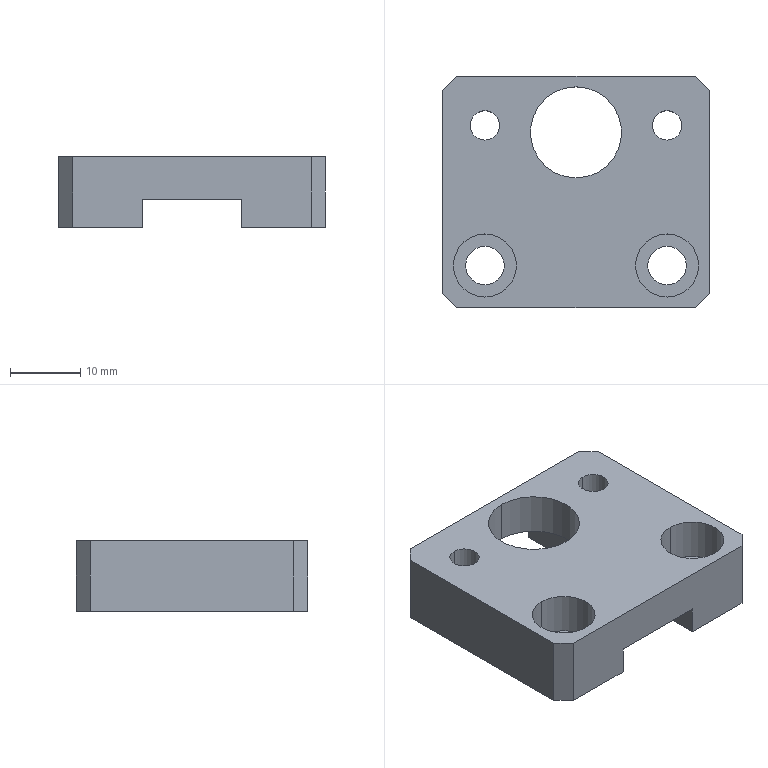Component | SolidWorks | DZ.KX.203-TC1505-30-09-01-05-19-1 | 1 solid | 30 faces | box 38 x 33 x 10 mm | volume 8585 mm3 | plane 16 | cylinder 14 | commonest cylinder face diameters 9 x4 5.5 x4 4.2 x4 13 x2
STEP:
#1=CARTESIAN_POINT('',(11.083,-23.614,0.8291));
#2=VERTEX_POINT('',#1);
#3=CARTESIAN_POINT('',(11.083,-23.26,0.8291));
#4=VERTEX_POINT('',#3);
#5=CARTESIAN_POINT('',(11.083,-23.437,0.8291));
#6=DIRECTION('',(0.,0.,1.));
#7=DIRECTION('',(0.,1.,0.));
#8=AXIS2_PLACEMENT_3D('',#5,#6,#7);
#9=CIRCLE('',#8,0.1772);
#10=EDGE_CURVE('',#2,#4,#9,.T.);
#11=ORIENTED_EDGE('',*,*,#10,.F.);
#12=CARTESIAN_POINT('',(11.083,-23.614,1.065));
#13=VERTEX_POINT('',#12);
#14=CARTESIAN_POINT('',(11.083,-23.614,1.065));
#15=DIRECTION('',(0.,0.,1.));
#16=VECTOR('',#15,39.37);
#17=LINE('',#14,#16);
#18=EDGE_CURVE('',#2,#13,#17,.T.);
#19=ORIENTED_EDGE('',*,*,#18,.T.);
#20=CARTESIAN_POINT('',(11.083,-23.26,1.065));
#21=VERTEX_POINT('',#20);
#22=CARTESIAN_POINT('',(11.083,-23.437,1.065));
#23=DIRECTION('',(0.,0.,1.));
#24=DIRECTION('',(0.,1.,0.));
#25=AXIS2_PLACEMENT_3D('',#22,#23,#24);
#26=CIRCLE('',#25,0.1772);
#27=EDGE_CURVE('',#13,#21,#26,.T.);
#28=ORIENTED_EDGE('',*,*,#27,.T.);
#29=CARTESIAN_POINT('',(11.083,-23.26,1.065));
#30=DIRECTION('',(0.,0.,1.));
#31=VECTOR('',#30,39.37);
#32=LINE('',#29,#31);
#33=EDGE_CURVE('',#4,#21,#32,.T.);
#34=ORIENTED_EDGE('',*,*,#33,.F.);
#35=EDGE_LOOP('',(#11,#19,#28,#34));
#36=FACE_OUTER_BOUND('',#35,.T.);
#37=CARTESIAN_POINT('',(11.083,-23.437,1.065));
#38=DIRECTION('',(0.,0.,1.));
#39=DIRECTION('',(0.,1.,0.));
#40=AXIS2_PLACEMENT_3D('',#37,#38,#39);
#41=CYLINDRICAL_SURFACE('',#40,0.1772);
#42=ADVANCED_FACE('',(#36),#41,.F.);
#43=CARTESIAN_POINT('',(11.083,-23.329,0.6716));
#44=VERTEX_POINT('',#43);
#45=CARTESIAN_POINT('',(11.083,-23.546,0.6716));
#46=VERTEX_POINT('',#45);
#47=CARTESIAN_POINT('',(11.083,-23.437,0.6716));
#48=DIRECTION('',(-0.,-0.,-1.));
#49=DIRECTION('',(0.,-1.,0.));
#50=AXIS2_PLACEMENT_3D('',#47,#48,#49);
#51=CIRCLE('',#50,0.1083);
#52=EDGE_CURVE('',#44,#46,#51,.T.);
#53=ORIENTED_EDGE('',*,*,#52,.T.);
#54=CARTESIAN_POINT('',(11.083,-23.546,0.8291));
#55=VERTEX_POINT('',#54);
#56=CARTESIAN_POINT('',(11.083,-23.546,1.065));
#57=DIRECTION('',(0.,0.,1.));
#58=VECTOR('',#57,39.37);
#59=LINE('',#56,#58);
#60=EDGE_CURVE('',#46,#55,#59,.T.);
#61=ORIENTED_EDGE('',*,*,#60,.T.);
#62=CARTESIAN_POINT('',(11.083,-23.329,0.8291));
#63=VERTEX_POINT('',#62);
#64=CARTESIAN_POINT('',(11.083,-23.437,0.8291));
#65=DIRECTION('',(0.,0.,1.));
#66=DIRECTION('',(0.,1.,0.));
#67=AXIS2_PLACEMENT_3D('',#64,#65,#66);
#68=CIRCLE('',#67,0.1083);
#69=EDGE_CURVE('',#55,#63,#68,.T.);
#70=ORIENTED_EDGE('',*,*,#69,.T.);
#71=CARTESIAN_POINT('',(11.083,-23.329,1.065));
#72=DIRECTION('',(0.,0.,1.));
#73=VECTOR('',#72,39.37);
#74=LINE('',#71,#73);
#75=EDGE_CURVE('',#44,#63,#74,.T.);
#76=ORIENTED_EDGE('',*,*,#75,.F.);
#77=EDGE_LOOP('',(#53,#61,#70,#76));
#78=FACE_OUTER_BOUND('',#77,.T.);
#79=CARTESIAN_POINT('',(11.083,-23.437,1.065));
#80=DIRECTION('',(0.,0.,1.));
#81=DIRECTION('',(0.,1.,0.));
#82=AXIS2_PLACEMENT_3D('',#79,#80,#81);
#83=CYLINDRICAL_SURFACE('',#82,0.1083);
#84=ADVANCED_FACE('',(#78),#83,.F.);
#85=CARTESIAN_POINT('',(12.106,-23.614,0.8291));
#86=VERTEX_POINT('',#85);
#87=CARTESIAN_POINT('',(12.106,-23.26,0.8291));
#88=VERTEX_POINT('',#87);
#89=CARTESIAN_POINT('',(12.106,-23.437,0.8291));
#90=DIRECTION('',(0.,0.,1.));
#91=DIRECTION('',(0.,1.,0.));
#92=AXIS2_PLACEMENT_3D('',#89,#90,#91);
#93=CIRCLE('',#92,0.1772);
#94=EDGE_CURVE('',#86,#88,#93,.T.);
#95=ORIENTED_EDGE('',*,*,#94,.F.);
#96=CARTESIAN_POINT('',(12.106,-23.614,1.065));
#97=VERTEX_POINT('',#96);
#98=CARTESIAN_POINT('',(12.106,-23.614,1.065));
#99=DIRECTION('',(0.,0.,1.));
#100=VECTOR('',#99,39.37);
#101=LINE('',#98,#100);
#102=EDGE_CURVE('',#86,#97,#101,.T.);
#103=ORIENTED_EDGE('',*,*,#102,.T.);
#104=CARTESIAN_POINT('',(12.106,-23.26,1.065));
#105=VERTEX_POINT('',#104);
#106=CARTESIAN_POINT('',(12.106,-23.437,1.065));
#107=DIRECTION('',(0.,0.,1.));
#108=DIRECTION('',(0.,1.,0.));
#109=AXIS2_PLACEMENT_3D('',#106,#107,#108);
#110=CIRCLE('',#109,0.1772);
#111=EDGE_CURVE('',#97,#105,#110,.T.);
#112=ORIENTED_EDGE('',*,*,#111,.T.);
#113=CARTESIAN_POINT('',(12.106,-23.26,1.065));
#114=DIRECTION('',(0.,0.,1.));
#115=VECTOR('',#114,39.37);
#116=LINE('',#113,#115);
#117=EDGE_CURVE('',#88,#105,#116,.T.);
#118=ORIENTED_EDGE('',*,*,#117,.F.);
#119=EDGE_LOOP('',(#95,#103,#112,#118));
#120=FACE_OUTER_BOUND('',#119,.T.);
#121=CARTESIAN_POINT('',(12.106,-23.437,1.065));
#122=DIRECTION('',(0.,0.,1.));
#123=DIRECTION('',(0.,1.,0.));
#124=AXIS2_PLACEMENT_3D('',#121,#122,#123);
#125=CYLINDRICAL_SURFACE('',#124,0.1772);
#126=ADVANCED_FACE('',(#120),#125,.F.);
#127=CARTESIAN_POINT('',(12.106,-23.329,0.6716));
#128=VERTEX_POINT('',#127);
#129=CARTESIAN_POINT('',(12.106,-23.546,0.6716));
#130=VERTEX_POINT('',#129);
#131=CARTESIAN_POINT('',(12.106,-23.437,0.6716));
#132=DIRECTION('',(-0.,-0.,-1.));
#133=DIRECTION('',(0.,-1.,0.));
#134=AXIS2_PLACEMENT_3D('',#131,#132,#133);
#135=CIRCLE('',#134,0.1083);
#136=EDGE_CURVE('',#128,#130,#135,.T.);
#137=ORIENTED_EDGE('',*,*,#136,.T.);
#138=CARTESIAN_POINT('',(12.106,-23.546,0.8291));
#139=VERTEX_POINT('',#138);
#140=CARTESIAN_POINT('',(12.106,-23.546,1.065));
#141=DIRECTION('',(0.,0.,1.));
#142=VECTOR('',#141,39.37);
#143=LINE('',#140,#142);
#144=EDGE_CURVE('',#130,#139,#143,.T.);
#145=ORIENTED_EDGE('',*,*,#144,.T.);
#146=CARTESIAN_POINT('',(12.106,-23.329,0.8291));
#147=VERTEX_POINT('',#146);
#148=CARTESIAN_POINT('',(12.106,-23.437,0.8291));
#149=DIRECTION('',(0.,0.,1.));
#150=DIRECTION('',(0.,1.,0.));
#151=AXIS2_PLACEMENT_3D('',#148,#149,#150);
#152=CIRCLE('',#151,0.1083);
#153=EDGE_CURVE('',#139,#147,#152,.T.);
#154=ORIENTED_EDGE('',*,*,#153,.T.);
#155=CARTESIAN_POINT('',(12.106,-23.329,1.065));
#156=DIRECTION('',(0.,0.,1.));
#157=VECTOR('',#156,39.37);
#158=LINE('',#155,#157);
#159=EDGE_CURVE('',#128,#147,#158,.T.);
#160=ORIENTED_EDGE('',*,*,#159,.F.);
#161=EDGE_LOOP('',(#137,#145,#154,#160));
#162=FACE_OUTER_BOUND('',#161,.T.);
#163=CARTESIAN_POINT('',(12.106,-23.437,1.065));
#164=DIRECTION('',(0.,0.,1.));
#165=DIRECTION('',(0.,1.,0.));
#166=AXIS2_PLACEMENT_3D('',#163,#164,#165);
#167=CYLINDRICAL_SURFACE('',#166,0.1083);
#168=ADVANCED_FACE('',(#162),#167,.F.);
#169=CARTESIAN_POINT('',(11.083,-22.567,1.065));
#170=VERTEX_POINT('',#169);
#171=CARTESIAN_POINT('',(11.083,-22.733,1.065));
#172=VERTEX_POINT('',#171);
#173=CARTESIAN_POINT('',(11.083,-22.65,1.065));
#174=DIRECTION('',(-0.,-0.,-1.));
#175=DIRECTION('',(0.,-1.,0.));
#176=AXIS2_PLACEMENT_3D('',#173,#174,#175);
#177=CIRCLE('',#176,0.08268);
#178=EDGE_CURVE('',#170,#172,#177,.T.);
#179=ORIENTED_EDGE('',*,*,#178,.F.);
#180=CARTESIAN_POINT('',(11.083,-22.567,0.6716));
#181=VERTEX_POINT('',#180);
#182=CARTESIAN_POINT('',(11.083,-22.567,0.6716));
#183=DIRECTION('',(-0.,-0.,-1.));
#184=VECTOR('',#183,39.37);
#185=LINE('',#182,#184);
#186=EDGE_CURVE('',#170,#181,#185,.T.);
#187=ORIENTED_EDGE('',*,*,#186,.T.);
#188=CARTESIAN_POINT('',(11.083,-22.733,0.6716));
#189=VERTEX_POINT('',#188);
#190=CARTESIAN_POINT('',(11.083,-22.65,0.6716));
#191=DIRECTION('',(-0.,-0.,-1.));
#192=DIRECTION('',(0.,-1.,0.));
#193=AXIS2_PLACEMENT_3D('',#190,#191,#192);
#194=CIRCLE('',#193,0.08268);
#195=EDGE_CURVE('',#181,#189,#194,.T.);
#196=ORIENTED_EDGE('',*,*,#195,.T.);
#197=CARTESIAN_POINT('',(11.083,-22.733,0.6716));
#198=DIRECTION('',(-0.,-0.,-1.));
#199=VECTOR('',#198,39.37);
#200=LINE('',#197,#199);
#201=EDGE_CURVE('',#172,#189,#200,.T.);
#202=ORIENTED_EDGE('',*,*,#201,.F.);
#203=EDGE_LOOP('',(#179,#187,#196,#202));
#204=FACE_OUTER_BOUND('',#203,.T.);
#205=CARTESIAN_POINT('',(11.083,-22.65,0.6716));
#206=DIRECTION('',(-0.,-0.,-1.));
#207=DIRECTION('',(0.,-1.,0.));
#208=AXIS2_PLACEMENT_3D('',#205,#206,#207);
#209=CYLINDRICAL_SURFACE('',#208,0.08268);
#210=ADVANCED_FACE('',(#204),#209,.F.);
#211=CARTESIAN_POINT('',(12.106,-22.567,1.065));
#212=VERTEX_POINT('',#211);
#213=CARTESIAN_POINT('',(12.106,-22.733,1.065));
#214=VERTEX_POINT('',#213);
#215=CARTESIAN_POINT('',(12.106,-22.65,1.065));
#216=DIRECTION('',(-0.,-0.,-1.));
#217=DIRECTION('',(0.,-1.,0.));
#218=AXIS2_PLACEMENT_3D('',#215,#216,#217);
#219=CIRCLE('',#218,0.08268);
#220=EDGE_CURVE('',#212,#214,#219,.T.);
#221=ORIENTED_EDGE('',*,*,#220,.F.);
#222=CARTESIAN_POINT('',(12.106,-22.567,0.6716));
#223=VERTEX_POINT('',#222);
#224=CARTESIAN_POINT('',(12.106,-22.567,0.6716));
#225=DIRECTION('',(-0.,-0.,-1.));
#226=VECTOR('',#225,39.37);
#227=LINE('',#224,#226);
#228=EDGE_CURVE('',#212,#223,#227,.T.);
#229=ORIENTED_EDGE('',*,*,#228,.T.);
#230=CARTESIAN_POINT('',(12.106,-22.733,0.6716));
#231=VERTEX_POINT('',#230);
#232=CARTESIAN_POINT('',(12.106,-22.65,0.6716));
#233=DIRECTION('',(-0.,-0.,-1.));
#234=DIRECTION('',(0.,-1.,0.));
#235=AXIS2_PLACEMENT_3D('',#232,#233,#234);
#236=CIRCLE('',#235,0.08268);
#237=EDGE_CURVE('',#223,#231,#236,.T.);
#238=ORIENTED_EDGE('',*,*,#237,.T.);
#239=CARTESIAN_POINT('',(12.106,-22.733,0.6716));
#240=DIRECTION('',(-0.,-0.,-1.));
#241=VECTOR('',#240,39.37);
#242=LINE('',#239,#241);
#243=EDGE_CURVE('',#214,#231,#242,.T.);
#244=ORIENTED_EDGE('',*,*,#243,.F.);
#245=EDGE_LOOP('',(#221,#229,#238,#244));
#246=FACE_OUTER_BOUND('',#245,.T.);
#247=CARTESIAN_POINT('',(12.106,-22.65,0.6716));
#248=DIRECTION('',(-0.,-0.,-1.));
#249=DIRECTION('',(0.,-1.,0.));
#250=AXIS2_PLACEMENT_3D('',#247,#248,#249);
#251=CYLINDRICAL_SURFACE('',#250,0.08268);
#252=ADVANCED_FACE('',(#246),#251,.F.);
#253=CARTESIAN_POINT('',(11.594,-22.433,0.8291));
#254=VERTEX_POINT('',#253);
#255=CARTESIAN_POINT('',(11.594,-22.945,0.8291));
#256=VERTEX_POINT('',#255);
#257=CARTESIAN_POINT('',(11.594,-22.689,0.8291));
#258=DIRECTION('',(-0.,-0.,-1.));
#259=DIRECTION('',(0.,-1.,0.));
#260=AXIS2_PLACEMENT_3D('',#257,#258,#259);
#261=CIRCLE('',#260,0.2559);
#262=EDGE_CURVE('',#254,#256,#261,.T.);
#263=ORIENTED_EDGE('',*,*,#262,.T.);
#264=CARTESIAN_POINT('',(11.594,-22.945,1.065));
#265=VERTEX_POINT('',#264);
#266=CARTESIAN_POINT('',(11.594,-22.945,0.6716));
#267=DIRECTION('',(0.,0.,1.));
#268=VECTOR('',#267,39.37);
#269=LINE('',#266,#268);
#270=EDGE_CURVE('',#256,#265,#269,.T.);
#271=ORIENTED_EDGE('',*,*,#270,.T.);
#272=CARTESIAN_POINT('',(11.594,-22.433,1.065));
#273=VERTEX_POINT('',#272);
#274=CARTESIAN_POINT('',(11.594,-22.689,1.065));
#275=DIRECTION('',(-0.,-0.,-1.));
#276=DIRECTION('',(0.,-1.,0.));
#277=AXIS2_PLACEMENT_3D('',#274,#275,#276);
#278=CIRCLE('',#277,0.2559);
#279=EDGE_CURVE('',#273,#265,#278,.T.);
#280=ORIENTED_EDGE('',*,*,#279,.F.);
#281=CARTESIAN_POINT('',(11.594,-22.433,0.6716));
#282=DIRECTION('',(0.,0.,1.));
#283=VECTOR('',#282,39.37);
#284=LINE('',#281,#283);
#285=EDGE_CURVE('',#254,#273,#284,.T.);
#286=ORIENTED_EDGE('',*,*,#285,.F.);
#287=EDGE_LOOP('',(#263,#271,#280,#286));
#288=FACE_OUTER_BOUND('',#287,.T.);
#289=CARTESIAN_POINT('',(11.594,-22.689,0.6716));
#290=DIRECTION('',(0.,0.,1.));
#291=DIRECTION('',(0.,1.,0.));
#292=AXIS2_PLACEMENT_3D('',#289,#290,#291);
#293=CYLINDRICAL_SURFACE('',#292,0.2559);
#294=ADVANCED_FACE('',(#288),#293,.F.);
#295=CARTESIAN_POINT('',(11.083,-23.437,1.065));
#296=DIRECTION('',(0.,0.,1.));
#297=DIRECTION('',(0.,1.,0.));
#298=AXIS2_PLACEMENT_3D('',#295,#296,#297);
#299=CIRCLE('',#298,0.1772);
#300=EDGE_CURVE('',#21,#13,#299,.T.);
#301=ORIENTED_EDGE('',*,*,#300,.F.);
#302=ORIENTED_EDGE('',*,*,#27,.F.);
#303=EDGE_LOOP('',(#301,#302));
#304=FACE_BOUND('',#303,.T.);
#305=CARTESIAN_POINT('',(12.106,-23.437,1.065));
#306=DIRECTION('',(0.,0.,1.));
#307=DIRECTION('',(0.,1.,0.));
#308=AXIS2_PLACEMENT_3D('',#305,#306,#307);
#309=CIRCLE('',#308,0.1772);
#310=EDGE_CURVE('',#105,#97,#309,.T.);
#311=ORIENTED_EDGE('',*,*,#310,.F.);
#312=ORIENTED_EDGE('',*,*,#111,.F.);
#313=EDGE_LOOP('',(#311,#312));
#314=FACE_BOUND('',#313,.T.);
#315=CARTESIAN_POINT('',(11.083,-22.65,1.065));
#316=DIRECTION('',(-0.,-0.,-1.));
#317=DIRECTION('',(0.,-1.,0.));
#318=AXIS2_PLACEMENT_3D('',#315,#316,#317);
#319=CIRCLE('',#318,0.08268);
#320=EDGE_CURVE('',#172,#170,#319,.T.);
#321=ORIENTED_EDGE('',*,*,#320,.T.);
#322=ORIENTED_EDGE('',*,*,#178,.T.);
#323=EDGE_LOOP('',(#321,#322));
#324=FACE_BOUND('',#323,.T.);
#325=CARTESIAN_POINT('',(12.106,-22.65,1.065));
#326=DIRECTION('',(-0.,-0.,-1.));
#327=DIRECTION('',(0.,-1.,0.));
#328=AXIS2_PLACEMENT_3D('',#325,#326,#327);
#329=CIRCLE('',#328,0.08268);
#330=EDGE_CURVE('',#214,#212,#329,.T.);
#331=ORIENTED_EDGE('',*,*,#330,.T.);
#332=ORIENTED_EDGE('',*,*,#220,.T.);
#333=EDGE_LOOP('',(#331,#332));
#334=FACE_BOUND('',#333,.T.);
#335=CARTESIAN_POINT('',(12.264,-23.674,1.065));
#336=VERTEX_POINT('',#335);
#337=CARTESIAN_POINT('',(10.925,-23.674,1.065));
#338=VERTEX_POINT('',#337);
#339=CARTESIAN_POINT('',(12.264,-23.674,1.065));
#340=DIRECTION('',(-1.,-0.,0.));
#341=VECTOR('',#340,39.37);
#342=LINE('',#339,#341);
#343=EDGE_CURVE('',#336,#338,#342,.T.);
#344=ORIENTED_EDGE('',*,*,#343,.F.);
#345=CARTESIAN_POINT('',(12.343,-23.595,1.065));
#346=VERTEX_POINT('',#345);
#347=CARTESIAN_POINT('',(12.264,-23.674,1.065));
#348=DIRECTION('',(0.7071,0.7071,-0.));
#349=VECTOR('',#348,39.37);
#350=LINE('',#347,#349);
#351=EDGE_CURVE('',#336,#346,#350,.T.);
#352=ORIENTED_EDGE('',*,*,#351,.T.);
#353=CARTESIAN_POINT('',(12.343,-22.453,1.065));
#354=VERTEX_POINT('',#353);
#355=CARTESIAN_POINT('',(12.343,-22.453,1.065));
#356=DIRECTION('',(0.,-1.,0.));
#357=VECTOR('',#356,39.37);
#358=LINE('',#355,#357);
#359=EDGE_CURVE('',#354,#346,#358,.T.);
#360=ORIENTED_EDGE('',*,*,#359,.F.);
#361=CARTESIAN_POINT('',(12.264,-22.374,1.065));
#362=VERTEX_POINT('',#361);
#363=CARTESIAN_POINT('',(12.264,-22.374,1.065));
#364=DIRECTION('',(0.7071,-0.7071,-0.));
#365=VECTOR('',#364,39.37);
#366=LINE('',#363,#365);
#367=EDGE_CURVE('',#362,#354,#366,.T.);
#368=ORIENTED_EDGE('',*,*,#367,.F.);
#369=CARTESIAN_POINT('',(10.925,-22.374,1.065));
#370=VERTEX_POINT('',#369);
#371=CARTESIAN_POINT('',(10.925,-22.374,1.065));
#372=DIRECTION('',(1.,0.,-0.));
#373=VECTOR('',#372,39.37);
#374=LINE('',#371,#373);
#375=EDGE_CURVE('',#370,#362,#374,.T.);
#376=ORIENTED_EDGE('',*,*,#375,.F.);
#377=CARTESIAN_POINT('',(10.846,-22.453,1.065));
#378=VERTEX_POINT('',#377);
#379=CARTESIAN_POINT('',(10.846,-22.453,1.065));
#380=DIRECTION('',(0.7071,0.7071,-0.));
#381=VECTOR('',#380,39.37);
#382=LINE('',#379,#381);
#383=EDGE_CURVE('',#378,#370,#382,.T.);
#384=ORIENTED_EDGE('',*,*,#383,.F.);
#385=CARTESIAN_POINT('',(10.846,-23.595,1.065));
#386=VERTEX_POINT('',#385);
#387=CARTESIAN_POINT('',(10.846,-22.925,1.065));
#388=DIRECTION('',(-0.,1.,-0.));
#389=VECTOR('',#388,39.37);
#390=LINE('',#387,#389);
#391=EDGE_CURVE('',#386,#378,#390,.T.);
#392=ORIENTED_EDGE('',*,*,#391,.F.);
#393=CARTESIAN_POINT('',(10.846,-23.595,1.065));
#394=DIRECTION('',(0.7071,-0.7071,-0.));
#395=VECTOR('',#394,39.37);
#396=LINE('',#393,#395);
#397=EDGE_CURVE('',#386,#338,#396,.T.);
#398=ORIENTED_EDGE('',*,*,#397,.T.);
#399=EDGE_LOOP('',(#344,#352,#360,#368,#376,#384,#392,#398));
#400=FACE_OUTER_BOUND('',#399,.T.);
#401=ORIENTED_EDGE('',*,*,#279,.T.);
#402=CARTESIAN_POINT('',(11.594,-22.689,1.065));
#403=DIRECTION('',(-0.,-0.,-1.));
#404=DIRECTION('',(0.,-1.,0.));
#405=AXIS2_PLACEMENT_3D('',#402,#403,#404);
#406=CIRCLE('',#405,0.2559);
#407=EDGE_CURVE('',#265,#273,#406,.T.);
#408=ORIENTED_EDGE('',*,*,#407,.T.);
#409=EDGE_LOOP('',(#401,#408));
#410=FACE_BOUND('',#409,.T.);
#411=CARTESIAN_POINT('',(12.343,-22.374,1.065));
#412=DIRECTION('',(-0.,-0.,-1.));
#413=DIRECTION('',(0.,-1.,0.));
#414=AXIS2_PLACEMENT_3D('',#411,#412,#413);
#415=PLANE('',#414);
#416=ADVANCED_FACE('',(#304,#314,#324,#334,#400,#410),#415,.F.);
#417=ORIENTED_EDGE('',*,*,#52,.F.);
#418=CARTESIAN_POINT('',(11.083,-23.437,0.6716));
#419=DIRECTION('',(-0.,-0.,-1.));
#420=DIRECTION('',(0.,-1.,0.));
#421=AXIS2_PLACEMENT_3D('',#418,#419,#420);
#422=CIRCLE('',#421,0.1083);
#423=EDGE_CURVE('',#46,#44,#422,.T.);
#424=ORIENTED_EDGE('',*,*,#423,.F.);
#425=EDGE_LOOP('',(#417,#424));
#426=FACE_BOUND('',#425,.T.);
#427=CARTESIAN_POINT('',(11.083,-22.65,0.6716));
#428=DIRECTION('',(-0.,-0.,-1.));
#429=DIRECTION('',(0.,-1.,0.));
#430=AXIS2_PLACEMENT_3D('',#427,#428,#429);
#431=CIRCLE('',#430,0.08268);
#432=EDGE_CURVE('',#189,#181,#431,.T.);
#433=ORIENTED_EDGE('',*,*,#432,.F.);
#434=ORIENTED_EDGE('',*,*,#195,.F.);
#435=EDGE_LOOP('',(#433,#434));
#436=FACE_BOUND('',#435,.T.);
#437=CARTESIAN_POINT('',(11.319,-23.674,0.6716));
#438=VERTEX_POINT('',#437);
#439=CARTESIAN_POINT('',(10.925,-23.674,0.6716));
#440=VERTEX_POINT('',#439);
#441=CARTESIAN_POINT('',(12.264,-23.674,0.6716));
#442=DIRECTION('',(-1.,-0.,0.));
#443=VECTOR('',#442,39.37);
#444=LINE('',#441,#443);
#445=EDGE_CURVE('',#438,#440,#444,.T.);
#446=ORIENTED_EDGE('',*,*,#445,.T.);
#447=CARTESIAN_POINT('',(10.846,-23.595,0.6716));
#448=VERTEX_POINT('',#447);
#449=CARTESIAN_POINT('',(10.984,-23.733,0.6716));
#450=DIRECTION('',(-0.7071,0.7071,0.));
#451=VECTOR('',#450,39.37);
#452=LINE('',#449,#451);
#453=EDGE_CURVE('',#440,#448,#452,.T.);
#454=ORIENTED_EDGE('',*,*,#453,.T.);
#455=CARTESIAN_POINT('',(10.846,-22.453,0.6716));
#456=VERTEX_POINT('',#455);
#457=CARTESIAN_POINT('',(10.846,-22.925,0.6716));
#458=DIRECTION('',(-0.,1.,-0.));
#459=VECTOR('',#458,39.37);
#460=LINE('',#457,#459);
#461=EDGE_CURVE('',#448,#456,#460,.T.);
#462=ORIENTED_EDGE('',*,*,#461,.T.);
#463=CARTESIAN_POINT('',(10.925,-22.374,0.6716));
#464=VERTEX_POINT('',#463);
#465=CARTESIAN_POINT('',(10.846,-22.453,0.6716));
#466=DIRECTION('',(0.7071,0.7071,-0.));
#467=VECTOR('',#466,39.37);
#468=LINE('',#465,#467);
#469=EDGE_CURVE('',#456,#464,#468,.T.);
#470=ORIENTED_EDGE('',*,*,#469,.T.);
#471=CARTESIAN_POINT('',(11.319,-22.374,0.6716));
#472=VERTEX_POINT('',#471);
#473=CARTESIAN_POINT('',(10.925,-22.374,0.6716));
#474=DIRECTION('',(1.,0.,-0.));
#475=VECTOR('',#474,39.37);
#476=LINE('',#473,#475);
#477=EDGE_CURVE('',#464,#472,#476,.T.);
#478=ORIENTED_EDGE('',*,*,#477,.T.);
#479=CARTESIAN_POINT('',(11.319,-22.374,0.6716));
#480=DIRECTION('',(0.,-1.,0.));
#481=VECTOR('',#480,39.37);
#482=LINE('',#479,#481);
#483=EDGE_CURVE('',#472,#438,#482,.T.);
#484=ORIENTED_EDGE('',*,*,#483,.T.);
#485=EDGE_LOOP('',(#446,#454,#462,#470,#478,#484));
#486=FACE_OUTER_BOUND('',#485,.T.);
#487=CARTESIAN_POINT('',(12.343,-22.374,0.6716));
#488=DIRECTION('',(-0.,-0.,-1.));
#489=DIRECTION('',(0.,-1.,0.));
#490=AXIS2_PLACEMENT_3D('',#487,#488,#489);
#491=PLANE('',#490);
#492=ADVANCED_FACE('',(#426,#436,#486),#491,.T.);
#493=ORIENTED_EDGE('',*,*,#136,.F.);
#494=CARTESIAN_POINT('',(12.106,-23.437,0.6716));
#495=DIRECTION('',(-0.,-0.,-1.));
#496=DIRECTION('',(0.,-1.,0.));
#497=AXIS2_PLACEMENT_3D('',#494,#495,#496);
#498=CIRCLE('',#497,0.1083);
#499=EDGE_CURVE('',#130,#128,#498,.T.);
#500=ORIENTED_EDGE('',*,*,#499,.F.);
#501=EDGE_LOOP('',(#493,#500));
#502=FACE_BOUND('',#501,.T.);
#503=CARTESIAN_POINT('',(12.106,-22.65,0.6716));
#504=DIRECTION('',(-0.,-0.,-1.));
#505=DIRECTION('',(0.,-1.,0.));
#506=AXIS2_PLACEMENT_3D('',#503,#504,#505);
#507=CIRCLE('',#506,0.08268);
#508=EDGE_CURVE('',#231,#223,#507,.T.);
#509=ORIENTED_EDGE('',*,*,#508,.F.);
#510=ORIENTED_EDGE('',*,*,#237,.F.);
#511=EDGE_LOOP('',(#509,#510));
#512=FACE_BOUND('',#511,.T.);
#513=CARTESIAN_POINT('',(12.343,-22.453,0.6716));
#514=VERTEX_POINT('',#513);
#515=CARTESIAN_POINT('',(12.343,-23.595,0.6716));
#516=VERTEX_POINT('',#515);
#517=CARTESIAN_POINT('',(12.343,-22.453,0.6716));
#518=DIRECTION('',(0.,-1.,0.));
#519=VECTOR('',#518,39.37);
#520=LINE('',#517,#519);
#521=EDGE_CURVE('',#514,#516,#520,.T.);
#522=ORIENTED_EDGE('',*,*,#521,.T.);
#523=CARTESIAN_POINT('',(12.264,-23.674,0.6716));
#524=VERTEX_POINT('',#523);
#525=CARTESIAN_POINT('',(12.953,-22.985,0.6716));
#526=DIRECTION('',(-0.7071,-0.7071,0.));
#527=VECTOR('',#526,39.37);
#528=LINE('',#525,#527);
#529=EDGE_CURVE('',#516,#524,#528,.T.);
#530=ORIENTED_EDGE('',*,*,#529,.T.);
#531=CARTESIAN_POINT('',(11.87,-23.674,0.6716));
#532=VERTEX_POINT('',#531);
#533=CARTESIAN_POINT('',(12.264,-23.674,0.6716));
#534=DIRECTION('',(-1.,-0.,0.));
#535=VECTOR('',#534,39.37);
#536=LINE('',#533,#535);
#537=EDGE_CURVE('',#524,#532,#536,.T.);
#538=ORIENTED_EDGE('',*,*,#537,.T.);
#539=CARTESIAN_POINT('',(11.87,-22.374,0.6716));
#540=VERTEX_POINT('',#539);
#541=CARTESIAN_POINT('',(11.87,-22.374,0.6716));
#542=DIRECTION('',(-0.,1.,-0.));
#543=VECTOR('',#542,39.37);
#544=LINE('',#541,#543);
#545=EDGE_CURVE('',#532,#540,#544,.T.);
#546=ORIENTED_EDGE('',*,*,#545,.T.);
#547=CARTESIAN_POINT('',(12.264,-22.374,0.6716));
#548=VERTEX_POINT('',#547);
#549=CARTESIAN_POINT('',(10.925,-22.374,0.6716));
#550=DIRECTION('',(1.,0.,-0.));
#551=VECTOR('',#550,39.37);
#552=LINE('',#549,#551);
#553=EDGE_CURVE('',#540,#548,#552,.T.);
#554=ORIENTED_EDGE('',*,*,#553,.T.);
#555=CARTESIAN_POINT('',(12.264,-22.374,0.6716));
#556=DIRECTION('',(0.7071,-0.7071,-0.));
#557=VECTOR('',#556,39.37);
#558=LINE('',#555,#557);
#559=EDGE_CURVE('',#548,#514,#558,.T.);
#560=ORIENTED_EDGE('',*,*,#559,.T.);
#561=EDGE_LOOP('',(#522,#530,#538,#546,#554,#560));
#562=FACE_OUTER_BOUND('',#561,.T.);
#563=CARTESIAN_POINT('',(12.343,-22.374,0.6716));
#564=DIRECTION('',(-0.,-0.,-1.));
#565=DIRECTION('',(0.,-1.,0.));
#566=AXIS2_PLACEMENT_3D('',#563,#564,#565);
#567=PLANE('',#566);
#568=ADVANCED_FACE('',(#502,#512,#562),#567,.T.);
#569=CARTESIAN_POINT('',(11.87,-22.374,0.8291));
#570=VERTEX_POINT('',#569);
#571=CARTESIAN_POINT('',(11.87,-22.374,0.5929));
#572=DIRECTION('',(0.,0.,1.));
#573=VECTOR('',#572,39.37);
#574=LINE('',#571,#573);
#575=EDGE_CURVE('',#540,#570,#574,.T.);
#576=ORIENTED_EDGE('',*,*,#575,.T.);
#577=CARTESIAN_POINT('',(11.319,-22.374,0.8291));
#578=VERTEX_POINT('',#577);
#579=CARTESIAN_POINT('',(11.87,-22.374,0.8291));
#580=DIRECTION('',(-1.,-0.,0.));
#581=VECTOR('',#580,39.37);
#582=LINE('',#579,#581);
#583=EDGE_CURVE('',#570,#578,#582,.T.);
#584=ORIENTED_EDGE('',*,*,#583,.T.);
#585=CARTESIAN_POINT('',(11.319,-22.374,0.8291));
#586=DIRECTION('',(-0.,-0.,-1.));
#587=VECTOR('',#586,39.37);
#588=LINE('',#585,#587);
#589=EDGE_CURVE('',#578,#472,#588,.T.);
#590=ORIENTED_EDGE('',*,*,#589,.T.);
#591=ORIENTED_EDGE('',*,*,#477,.F.);
#592=CARTESIAN_POINT('',(10.925,-22.374,0.6716));
#593=DIRECTION('',(0.,0.,1.));
#594=VECTOR('',#593,39.37);
#595=LINE('',#592,#594);
#596=EDGE_CURVE('',#464,#370,#595,.T.);
#597=ORIENTED_EDGE('',*,*,#596,.T.);
#598=ORIENTED_EDGE('',*,*,#375,.T.);
#599=CARTESIAN_POINT('',(12.264,-22.374,0.6716));
#600=DIRECTION('',(0.,0.,1.));
#601=VECTOR('',#600,39.37);
#602=LINE('',#599,#601);
#603=EDGE_CURVE('',#548,#362,#602,.T.);
#604=ORIENTED_EDGE('',*,*,#603,.F.);
#605=ORIENTED_EDGE('',*,*,#553,.F.);
#606=EDGE_LOOP('',(#576,#584,#590,#591,#597,#598,#604,#605));
#607=FACE_OUTER_BOUND('',#606,.T.);
#608=CARTESIAN_POINT('',(10.925,-22.374,0.6716));
#609=DIRECTION('',(0.,-1.,0.));
#610=DIRECTION('',(0.,0.,1.));
#611=AXIS2_PLACEMENT_3D('',#608,#609,#610);
#612=PLANE('',#611);
#613=ADVANCED_FACE('',(#607),#612,.F.);
#614=ORIENTED_EDGE('',*,*,#537,.F.);
#615=CARTESIAN_POINT('',(12.264,-23.674,0.6716));
#616=DIRECTION('',(0.,0.,1.));
#617=VECTOR('',#616,39.37);
#618=LINE('',#615,#617);
#619=EDGE_CURVE('',#524,#336,#618,.T.);
#620=ORIENTED_EDGE('',*,*,#619,.T.);
#621=ORIENTED_EDGE('',*,*,#343,.T.);
#622=CARTESIAN_POINT('',(10.925,-23.674,0.6716));
#623=DIRECTION('',(-0.,-0.,-1.));
#624=VECTOR('',#623,39.37);
#625=LINE('',#622,#624);
#626=EDGE_CURVE('',#338,#440,#625,.T.);
#627=ORIENTED_EDGE('',*,*,#626,.T.);
#628=ORIENTED_EDGE('',*,*,#445,.F.);
#629=CARTESIAN_POINT('',(11.319,-23.674,0.8291));
#630=VERTEX_POINT('',#629);
#631=CARTESIAN_POINT('',(11.319,-23.674,0.6716));
#632=DIRECTION('',(-0.,-0.,-1.));
#633=VECTOR('',#632,39.37);
#634=LINE('',#631,#633);
#635=EDGE_CURVE('',#630,#438,#634,.T.);
#636=ORIENTED_EDGE('',*,*,#635,.F.);
#637=CARTESIAN_POINT('',(11.87,-23.674,0.8291));
#638=VERTEX_POINT('',#637);
#639=CARTESIAN_POINT('',(12.264,-23.674,0.8291));
#640=DIRECTION('',(-1.,-0.,0.));
#641=VECTOR('',#640,39.37);
#642=LINE('',#639,#641);
#643=EDGE_CURVE('',#638,#630,#642,.T.);
#644=ORIENTED_EDGE('',*,*,#643,.F.);
#645=CARTESIAN_POINT('',(11.87,-23.674,0.6716));
#646=DIRECTION('',(0.,0.,1.));
#647=VECTOR('',#646,39.37);
#648=LINE('',#645,#647);
#649=EDGE_CURVE('',#532,#638,#648,.T.);
#650=ORIENTED_EDGE('',*,*,#649,.F.);
#651=EDGE_LOOP('',(#614,#620,#621,#627,#628,#636,#644,#650));
#652=FACE_OUTER_BOUND('',#651,.T.);
#653=CARTESIAN_POINT('',(12.264,-23.674,0.6716));
#654=DIRECTION('',(-0.,1.,-0.));
#655=DIRECTION('',(-0.,-0.,-1.));
#656=AXIS2_PLACEMENT_3D('',#653,#654,#655);
#657=PLANE('',#656);
#658=ADVANCED_FACE('',(#652),#657,.F.);
#659=ORIENTED_EDGE('',*,*,#270,.F.);
#660=CARTESIAN_POINT('',(11.594,-22.689,0.8291));
#661=DIRECTION('',(-0.,-0.,-1.));
#662=DIRECTION('',(0.,-1.,0.));
#663=AXIS2_PLACEMENT_3D('',#660,#661,#662);
#664=CIRCLE('',#663,0.2559);
#665=EDGE_CURVE('',#256,#254,#664,.T.);
#666=ORIENTED_EDGE('',*,*,#665,.T.);
#667=ORIENTED_EDGE('',*,*,#285,.T.);
#668=ORIENTED_EDGE('',*,*,#407,.F.);
#669=EDGE_LOOP('',(#659,#666,#667,#668));
#670=FACE_OUTER_BOUND('',#669,.T.);
#671=CARTESIAN_POINT('',(11.594,-22.689,0.6716));
#672=DIRECTION('',(0.,0.,1.));
#673=DIRECTION('',(0.,1.,0.));
#674=AXIS2_PLACEMENT_3D('',#671,#672,#673);
#675=CYLINDRICAL_SURFACE('',#674,0.2559);
#676=ADVANCED_FACE('',(#670),#675,.F.);
#677=ORIENTED_EDGE('',*,*,#383,.T.);
#678=ORIENTED_EDGE('',*,*,#596,.F.);
#679=ORIENTED_EDGE('',*,*,#469,.F.);
#680=CARTESIAN_POINT('',(10.846,-22.453,0.6716));
#681=DIRECTION('',(0.,0.,1.));
#682=VECTOR('',#681,39.37);
#683=LINE('',#680,#682);
#684=EDGE_CURVE('',#456,#378,#683,.T.);
#685=ORIENTED_EDGE('',*,*,#684,.T.);
#686=EDGE_LOOP('',(#677,#678,#679,#685));
#687=FACE_OUTER_BOUND('',#686,.T.);
#688=CARTESIAN_POINT('',(10.846,-22.453,0.6716));
#689=DIRECTION('',(0.7071,-0.7071,-0.));
#690=DIRECTION('',(-0.7071,-0.7071,0.));
#691=AXIS2_PLACEMENT_3D('',#688,#689,#690);
#692=PLANE('',#691);
#693=ADVANCED_FACE('',(#687),#692,.F.);
#694=ORIENTED_EDGE('',*,*,#367,.T.);
#695=CARTESIAN_POINT('',(12.343,-22.453,0.6716));
#696=DIRECTION('',(0.,0.,1.));
#697=VECTOR('',#696,39.37);
#698=LINE('',#695,#697);
#699=EDGE_CURVE('',#514,#354,#698,.T.);
#700=ORIENTED_EDGE('',*,*,#699,.F.);
#701=ORIENTED_EDGE('',*,*,#559,.F.);
#702=ORIENTED_EDGE('',*,*,#603,.T.);
#703=EDGE_LOOP('',(#694,#700,#701,#702));
#704=FACE_OUTER_BOUND('',#703,.T.);
#705=CARTESIAN_POINT('',(12.264,-22.374,0.6716));
#706=DIRECTION('',(-0.7071,-0.7071,0.));
#707=DIRECTION('',(-0.7071,0.7071,0.));
#708=AXIS2_PLACEMENT_3D('',#705,#706,#707);
#709=PLANE('',#708);
#710=ADVANCED_FACE('',(#704),#709,.F.);
#711=ORIENTED_EDGE('',*,*,#359,.T.);
#712=CARTESIAN_POINT('',(12.343,-23.595,0.6716));
#713=DIRECTION('',(-0.,-0.,-1.));
#714=VECTOR('',#713,39.37);
#715=LINE('',#712,#714);
#716=EDGE_CURVE('',#346,#516,#715,.T.);
#717=ORIENTED_EDGE('',*,*,#716,.T.);
#718=ORIENTED_EDGE('',*,*,#521,.F.);
#719=ORIENTED_EDGE('',*,*,#699,.T.);
#720=EDGE_LOOP('',(#711,#717,#718,#719));
#721=FACE_OUTER_BOUND('',#720,.T.);
#722=CARTESIAN_POINT('',(12.343,-22.453,0.6716));
#723=DIRECTION('',(-1.,-0.,0.));
#724=DIRECTION('',(-0.,-0.,-1.));
#725=AXIS2_PLACEMENT_3D('',#722,#723,#724);
#726=PLANE('',#725);
#727=ADVANCED_FACE('',(#721),#726,.F.);
#728=ORIENTED_EDGE('',*,*,#461,.F.);
#729=CARTESIAN_POINT('',(10.846,-23.595,0.6716));
#730=DIRECTION('',(0.,0.,1.));
#731=VECTOR('',#730,39.37);
#732=LINE('',#729,#731);
#733=EDGE_CURVE('',#448,#386,#732,.T.);
#734=ORIENTED_EDGE('',*,*,#733,.T.);
#735=ORIENTED_EDGE('',*,*,#391,.T.);
#736=ORIENTED_EDGE('',*,*,#684,.F.);
#737=EDGE_LOOP('',(#728,#734,#735,#736));
#738=FACE_OUTER_BOUND('',#737,.T.);
#739=CARTESIAN_POINT('',(10.846,-22.925,0.6716));
#740=DIRECTION('',(1.,0.,-0.));
#741=DIRECTION('',(0.,0.,1.));
#742=AXIS2_PLACEMENT_3D('',#739,#740,#741);
#743=PLANE('',#742);
#744=ADVANCED_FACE('',(#738),#743,.F.);
#745=ORIENTED_EDGE('',*,*,#649,.T.);
#746=CARTESIAN_POINT('',(11.87,-23.004,0.8291));
#747=DIRECTION('',(-0.,1.,-0.));
#748=VECTOR('',#747,39.37);
#749=LINE('',#746,#748);
#750=EDGE_CURVE('',#638,#570,#749,.T.);
#751=ORIENTED_EDGE('',*,*,#750,.T.);
#752=ORIENTED_EDGE('',*,*,#575,.F.);
#753=ORIENTED_EDGE('',*,*,#545,.F.);
#754=EDGE_LOOP('',(#745,#751,#752,#753));
#755=FACE_OUTER_BOUND('',#754,.T.);
#756=CARTESIAN_POINT('',(11.87,-23.004,0.5929));
#757=DIRECTION('',(-1.,-0.,0.));
#758=DIRECTION('',(-0.,-0.,-1.));
#759=AXIS2_PLACEMENT_3D('',#756,#757,#758);
#760=PLANE('',#759);
#761=ADVANCED_FACE('',(#755),#760,.T.);
#762=ORIENTED_EDGE('',*,*,#262,.F.);
#763=ORIENTED_EDGE('',*,*,#665,.F.);
#764=EDGE_LOOP('',(#762,#763));
#765=FACE_BOUND('',#764,.T.);
#766=ORIENTED_EDGE('',*,*,#583,.F.);
#767=ORIENTED_EDGE('',*,*,#750,.F.);
#768=ORIENTED_EDGE('',*,*,#643,.T.);
#769=CARTESIAN_POINT('',(11.319,-23.004,0.8291));
#770=DIRECTION('',(-0.,1.,-0.));
#771=VECTOR('',#770,39.37);
#772=LINE('',#769,#771);
#773=EDGE_CURVE('',#630,#578,#772,.T.);
#774=ORIENTED_EDGE('',*,*,#773,.T.);
#775=EDGE_LOOP('',(#766,#767,#768,#774));
#776=FACE_OUTER_BOUND('',#775,.T.);
#777=CARTESIAN_POINT('',(11.87,-23.004,0.8291));
#778=DIRECTION('',(-0.,-0.,-1.));
#779=DIRECTION('',(0.,-1.,0.));
#780=AXIS2_PLACEMENT_3D('',#777,#778,#779);
#781=PLANE('',#780);
#782=ADVANCED_FACE('',(#765,#776),#781,.T.);
#783=ORIENTED_EDGE('',*,*,#589,.F.);
#784=ORIENTED_EDGE('',*,*,#773,.F.);
#785=ORIENTED_EDGE('',*,*,#635,.T.);
#786=ORIENTED_EDGE('',*,*,#483,.F.);
#787=EDGE_LOOP('',(#783,#784,#785,#786));
#788=FACE_OUTER_BOUND('',#787,.T.);
#789=CARTESIAN_POINT('',(11.319,-23.004,0.8291));
#790=DIRECTION('',(1.,0.,-0.));
#791=DIRECTION('',(0.,0.,1.));
#792=AXIS2_PLACEMENT_3D('',#789,#790,#791);
#793=PLANE('',#792);
#794=ADVANCED_FACE('',(#788),#793,.T.);
#795=ORIENTED_EDGE('',*,*,#529,.F.);
#796=ORIENTED_EDGE('',*,*,#716,.F.);
#797=ORIENTED_EDGE('',*,*,#351,.F.);
#798=ORIENTED_EDGE('',*,*,#619,.F.);
#799=EDGE_LOOP('',(#795,#796,#797,#798));
#800=FACE_OUTER_BOUND('',#799,.T.);
#801=CARTESIAN_POINT('',(12.264,-23.674,0.6716));
#802=DIRECTION('',(-0.7071,0.7071,0.));
#803=DIRECTION('',(0.,0.,1.));
#804=AXIS2_PLACEMENT_3D('',#801,#802,#803);
#805=PLANE('',#804);
#806=ADVANCED_FACE('',(#800),#805,.F.);
#807=ORIENTED_EDGE('',*,*,#453,.F.);
#808=ORIENTED_EDGE('',*,*,#626,.F.);
#809=ORIENTED_EDGE('',*,*,#397,.F.);
#810=ORIENTED_EDGE('',*,*,#733,.F.);
#811=EDGE_LOOP('',(#807,#808,#809,#810));
#812=FACE_OUTER_BOUND('',#811,.T.);
#813=CARTESIAN_POINT('',(10.846,-23.595,0.6716));
#814=DIRECTION('',(0.7071,0.7071,-0.));
#815=DIRECTION('',(0.,0.,1.));
#816=AXIS2_PLACEMENT_3D('',#813,#814,#815);
#817=PLANE('',#816);
#818=ADVANCED_FACE('',(#812),#817,.F.);
#819=ORIENTED_EDGE('',*,*,#228,.F.);
#820=ORIENTED_EDGE('',*,*,#330,.F.);
#821=ORIENTED_EDGE('',*,*,#243,.T.);
#822=ORIENTED_EDGE('',*,*,#508,.T.);
#823=EDGE_LOOP('',(#819,#820,#821,#822));
#824=FACE_OUTER_BOUND('',#823,.T.);
#825=CARTESIAN_POINT('',(12.106,-22.65,0.6716));
#826=DIRECTION('',(-0.,-0.,-1.));
#827=DIRECTION('',(0.,-1.,0.));
#828=AXIS2_PLACEMENT_3D('',#825,#826,#827);
#829=CYLINDRICAL_SURFACE('',#828,0.08268);
#830=ADVANCED_FACE('',(#824),#829,.F.);
#831=ORIENTED_EDGE('',*,*,#186,.F.);
#832=ORIENTED_EDGE('',*,*,#320,.F.);
#833=ORIENTED_EDGE('',*,*,#201,.T.);
#834=ORIENTED_EDGE('',*,*,#432,.T.);
#835=EDGE_LOOP('',(#831,#832,#833,#834));
#836=FACE_OUTER_BOUND('',#835,.T.);
#837=CARTESIAN_POINT('',(11.083,-22.65,0.6716));
#838=DIRECTION('',(-0.,-0.,-1.));
#839=DIRECTION('',(0.,-1.,0.));
#840=AXIS2_PLACEMENT_3D('',#837,#838,#839);
#841=CYLINDRICAL_SURFACE('',#840,0.08268);
#842=ADVANCED_FACE('',(#836),#841,.F.);
#843=ORIENTED_EDGE('',*,*,#144,.F.);
#844=ORIENTED_EDGE('',*,*,#499,.T.);
#845=ORIENTED_EDGE('',*,*,#159,.T.);
#846=CARTESIAN_POINT('',(12.106,-23.437,0.8291));
#847=DIRECTION('',(0.,0.,1.));
#848=DIRECTION('',(0.,1.,0.));
#849=AXIS2_PLACEMENT_3D('',#846,#847,#848);
#850=CIRCLE('',#849,0.1083);
#851=EDGE_CURVE('',#147,#139,#850,.T.);
#852=ORIENTED_EDGE('',*,*,#851,.T.);
#853=EDGE_LOOP('',(#843,#844,#845,#852));
#854=FACE_OUTER_BOUND('',#853,.T.);
#855=CARTESIAN_POINT('',(12.106,-23.437,1.065));
#856=DIRECTION('',(0.,0.,1.));
#857=DIRECTION('',(0.,1.,0.));
#858=AXIS2_PLACEMENT_3D('',#855,#856,#857);
#859=CYLINDRICAL_SURFACE('',#858,0.1083);
#860=ADVANCED_FACE('',(#854),#859,.F.);
#861=ORIENTED_EDGE('',*,*,#851,.F.);
#862=ORIENTED_EDGE('',*,*,#153,.F.);
#863=EDGE_LOOP('',(#861,#862));
#864=FACE_BOUND('',#863,.T.);
#865=CARTESIAN_POINT('',(12.106,-23.437,0.8291));
#866=DIRECTION('',(0.,0.,1.));
#867=DIRECTION('',(0.,1.,0.));
#868=AXIS2_PLACEMENT_3D('',#865,#866,#867);
#869=CIRCLE('',#868,0.1772);
#870=EDGE_CURVE('',#88,#86,#869,.T.);
#871=ORIENTED_EDGE('',*,*,#870,.T.);
#872=ORIENTED_EDGE('',*,*,#94,.T.);
#873=EDGE_LOOP('',(#871,#872));
#874=FACE_OUTER_BOUND('',#873,.T.);
#875=CARTESIAN_POINT('',(12.018,-23.437,0.8291));
#876=DIRECTION('',(0.,0.,1.));
#877=DIRECTION('',(-0.,1.,-0.));
#878=AXIS2_PLACEMENT_3D('',#875,#876,#877);
#879=PLANE('',#878);
#880=ADVANCED_FACE('',(#864,#874),#879,.T.);
#881=ORIENTED_EDGE('',*,*,#102,.F.);
#882=ORIENTED_EDGE('',*,*,#870,.F.);
#883=ORIENTED_EDGE('',*,*,#117,.T.);
#884=ORIENTED_EDGE('',*,*,#310,.T.);
#885=EDGE_LOOP('',(#881,#882,#883,#884));
#886=FACE_OUTER_BOUND('',#885,.T.);
#887=CARTESIAN_POINT('',(12.106,-23.437,1.065));
#888=DIRECTION('',(0.,0.,1.));
#889=DIRECTION('',(0.,1.,0.));
#890=AXIS2_PLACEMENT_3D('',#887,#888,#889);
#891=CYLINDRICAL_SURFACE('',#890,0.1772);
#892=ADVANCED_FACE('',(#886),#891,.F.);
#893=ORIENTED_EDGE('',*,*,#60,.F.);
#894=ORIENTED_EDGE('',*,*,#423,.T.);
#895=ORIENTED_EDGE('',*,*,#75,.T.);
#896=CARTESIAN_POINT('',(11.083,-23.437,0.8291));
#897=DIRECTION('',(0.,0.,1.));
#898=DIRECTION('',(0.,1.,0.));
#899=AXIS2_PLACEMENT_3D('',#896,#897,#898);
#900=CIRCLE('',#899,0.1083);
#901=EDGE_CURVE('',#63,#55,#900,.T.);
#902=ORIENTED_EDGE('',*,*,#901,.T.);
#903=EDGE_LOOP('',(#893,#894,#895,#902));
#904=FACE_OUTER_BOUND('',#903,.T.);
#905=CARTESIAN_POINT('',(11.083,-23.437,1.065));
#906=DIRECTION('',(0.,0.,1.));
#907=DIRECTION('',(0.,1.,0.));
#908=AXIS2_PLACEMENT_3D('',#905,#906,#907);
#909=CYLINDRICAL_SURFACE('',#908,0.1083);
#910=ADVANCED_FACE('',(#904),#909,.F.);
#911=ORIENTED_EDGE('',*,*,#18,.F.);
#912=CARTESIAN_POINT('',(11.083,-23.437,0.8291));
#913=DIRECTION('',(0.,0.,1.));
#914=DIRECTION('',(0.,1.,0.));
#915=AXIS2_PLACEMENT_3D('',#912,#913,#914);
#916=CIRCLE('',#915,0.1772);
#917=EDGE_CURVE('',#4,#2,#916,.T.);
#918=ORIENTED_EDGE('',*,*,#917,.F.);
#919=ORIENTED_EDGE('',*,*,#33,.T.);
#920=ORIENTED_EDGE('',*,*,#300,.T.);
#921=EDGE_LOOP('',(#911,#918,#919,#920));
#922=FACE_OUTER_BOUND('',#921,.T.);
#923=CARTESIAN_POINT('',(11.083,-23.437,1.065));
#924=DIRECTION('',(0.,0.,1.));
#925=DIRECTION('',(0.,1.,0.));
#926=AXIS2_PLACEMENT_3D('',#923,#924,#925);
#927=CYLINDRICAL_SURFACE('',#926,0.1772);
#928=ADVANCED_FACE('',(#922),#927,.F.);
#929=ORIENTED_EDGE('',*,*,#901,.F.);
#930=ORIENTED_EDGE('',*,*,#69,.F.);
#931=EDGE_LOOP('',(#929,#930));
#932=FACE_BOUND('',#931,.T.);
#933=ORIENTED_EDGE('',*,*,#917,.T.);
#934=ORIENTED_EDGE('',*,*,#10,.T.);
#935=EDGE_LOOP('',(#933,#934));
#936=FACE_OUTER_BOUND('',#935,.T.);
#937=CARTESIAN_POINT('',(10.994,-23.437,0.8291));
#938=DIRECTION('',(0.,0.,1.));
#939=DIRECTION('',(-0.,1.,-0.));
#940=AXIS2_PLACEMENT_3D('',#937,#938,#939);
#941=PLANE('',#940);
#942=ADVANCED_FACE('',(#932,#936),#941,.T.);
#943=CLOSED_SHELL('',(#42,#84,#126,#168,#210,#252,#294,#416,#492,#568,#613,#658,#676,#693,#710,#727,#744,#761,#782,#794,#806,#818,#830,#842,#860,#880,#892,#910,#928,#942));
#944=MANIFOLD_SOLID_BREP('',#943);
#945=CARTESIAN_POINT('',(0.,0.,0.));
#946=DIRECTION('',(0.,0.,1.));
#947=DIRECTION('',(1.,0.,0.));
#948=AXIS2_PLACEMENT_3D('',#945,#946,#947);
#949=(LENGTH_UNIT()NAMED_UNIT(*)SI_UNIT($,.METRE.));
#950=LENGTH_MEASURE_WITH_UNIT(LENGTH_MEASURE(0.0254),#949);
#951=DIMENSIONAL_EXPONENTS(1.,0.,0.,0.,0.,0.,0.);
#952=(CONVERSION_BASED_UNIT('',#950)LENGTH_UNIT()NAMED_UNIT(#951));
#953=UNCERTAINTY_MEASURE_WITH_UNIT(LENGTH_MEASURE(0.00001),#952,'','');
#954=(NAMED_UNIT(*)PLANE_ANGLE_UNIT()SI_UNIT($,.RADIAN.));
#955=(NAMED_UNIT(*)SI_UNIT($,.STERADIAN.)SOLID_ANGLE_UNIT());
#956=(GEOMETRIC_REPRESENTATION_CONTEXT(3)GLOBAL_UNCERTAINTY_ASSIGNED_CONTEXT((#953))GLOBAL_UNIT_ASSIGNED_CONTEXT((#952,#954,#955))REPRESENTATION_CONTEXT('',''));
#957=ADVANCED_BREP_SHAPE_REPRESENTATION('',(#944,#948),#956);
#958=COLOUR_RGB('',0.7922,0.8196,0.9333);
#959=FILL_AREA_STYLE_COLOUR('',#958);
#960=FILL_AREA_STYLE('',(#959));
#961=SURFACE_STYLE_FILL_AREA(#960);
#962=SURFACE_SIDE_STYLE('',(#961));
#963=SURFACE_STYLE_USAGE(.BOTH.,#962);
#964=PRESENTATION_STYLE_ASSIGNMENT((#963));
#965=STYLED_ITEM('',(#964),#944);
#966=(LENGTH_UNIT()NAMED_UNIT(*)SI_UNIT($,.METRE.));
#967=LENGTH_MEASURE_WITH_UNIT(LENGTH_MEASURE(0.0254),#966);
#968=DIMENSIONAL_EXPONENTS(1.,0.,0.,0.,0.,0.,0.);
#969=(CONVERSION_BASED_UNIT('',#967)LENGTH_UNIT()NAMED_UNIT(#968));
#970=UNCERTAINTY_MEASURE_WITH_UNIT(LENGTH_MEASURE(0.00001),#969,'','');
#971=(NAMED_UNIT(*)PLANE_ANGLE_UNIT()SI_UNIT($,.RADIAN.));
#972=(NAMED_UNIT(*)SI_UNIT($,.STERADIAN.)SOLID_ANGLE_UNIT());
#973=(GEOMETRIC_REPRESENTATION_CONTEXT(3)GLOBAL_UNCERTAINTY_ASSIGNED_CONTEXT((#970))GLOBAL_UNIT_ASSIGNED_CONTEXT((#969,#971,#972))REPRESENTATION_CONTEXT('',''));
#974=MECHANICAL_DESIGN_GEOMETRIC_PRESENTATION_REPRESENTATION('',(#965),#973);
#975=PRESENTATION_LAYER_ASSIGNMENT('','',(#965));